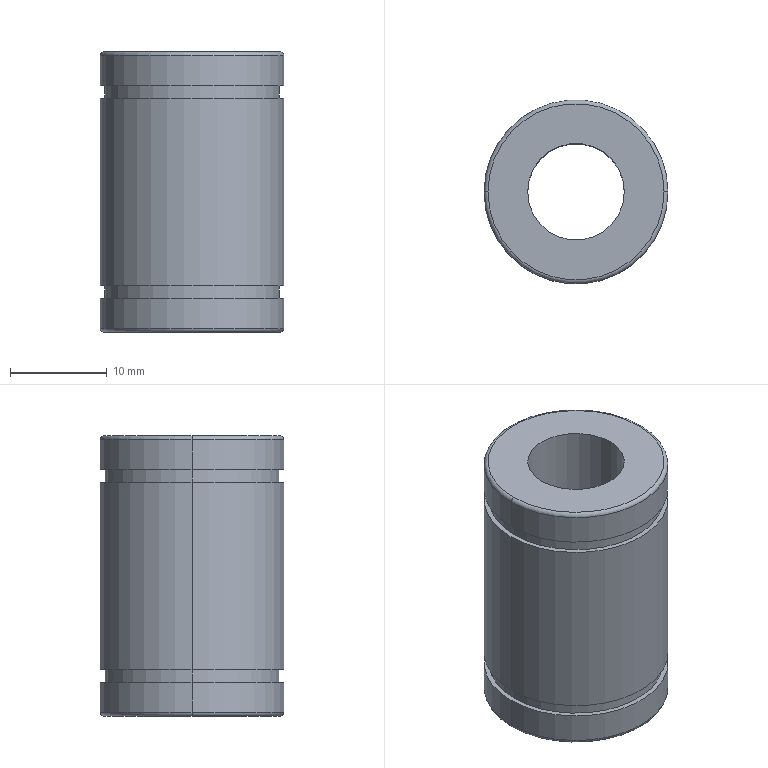Component | SolidWorks | LMU_N10-10 | 1 solid | 22 faces | box 19 x 19 x 29 mm | volume 5865 mm3 | cylinder 12 | plane 6 | torus 4 | commonest cylinder face diameters 19 x6 18 x4 10 x2
build123d program:
from build123d import *


with BuildPart() as part:
    # Sketch1 → Revolve1 (revolve)
    with BuildSketch(Plane.XY, mode=Mode.PRIVATE) as revolve1_sk:
        with BuildLine():
            Line((0, 9.1), (0, 5))
            Line((0, 5), (29, 5))
            Line((29, 5), (29, 9.1))
            ThreePointArc((29, 9.1), (28.883, 9.383), (28.6, 9.5))
            Line((28.6, 9.5), (25.5, 9.5))
            Line((25.5, 9.5), (25.5, 9))
            Line((25.5, 9), (24.2, 9))
            Line((24.2, 9), (24.2, 9.5))
            Line((24.2, 9.5), (4.8, 9.5))
            Line((4.8, 9.5), (4.8, 9))
            Line((4.8, 9), (3.5, 9))
            Line((3.5, 9), (3.5, 9.5))
            Line((3.5, 9.5), (0.4, 9.5))
            ThreePointArc((0.4, 9.5), (0.1172, 9.383), (0, 9.1))
        make_face()
    revolve(revolve1_sk.sketch.rotate(Axis((29, 0, 0), (-1, 0, 0)), 270), axis=Axis((29, 0, 0), (-1, 0, 0)))


solid = part.part

# Placed as in the assembly
solid = solid.moved(Location((860.265, 384.385, -295.193), (0, 90, 0)))
STEP:
#1=COLOUR_RGB('',0.7922,0.8196,0.9333);
#2=FILL_AREA_STYLE_COLOUR('',#1);
#3=FILL_AREA_STYLE('',(#2));
#4=SURFACE_STYLE_FILL_AREA(#3);
#5=SURFACE_SIDE_STYLE('',(#4));
#6=SURFACE_STYLE_USAGE(.BOTH.,#5);
#7=PRESENTATION_STYLE_ASSIGNMENT((#6));
#8=CARTESIAN_POINT('',(33.495,15.133,-12.626));
#9=VERTEX_POINT('',#8);
#10=CARTESIAN_POINT('',(34.243,15.133,-12.626));
#11=VERTEX_POINT('',#10);
#12=CARTESIAN_POINT('',(33.869,15.133,-12.626));
#13=DIRECTION('',(-0.00002551,-0.,-1.));
#14=DIRECTION('',(-1.,0.,0.00002551));
#15=AXIS2_PLACEMENT_3D('',#12,#13,#14);
#16=CIRCLE('',#15,0.374);
#17=EDGE_CURVE('',#9,#11,#16,.T.);
#18=ORIENTED_EDGE('',*,*,#17,.T.);
#19=CARTESIAN_POINT('',(34.243,15.133,-12.748));
#20=VERTEX_POINT('',#19);
#21=CARTESIAN_POINT('',(34.243,15.133,-11.622));
#22=DIRECTION('',(-0.00002551,-0.,-1.));
#23=VECTOR('',#22,39.37);
#24=LINE('',#21,#23);
#25=EDGE_CURVE('',#11,#20,#24,.T.);
#26=ORIENTED_EDGE('',*,*,#25,.T.);
#27=CARTESIAN_POINT('',(33.495,15.133,-12.748));
#28=VERTEX_POINT('',#27);
#29=CARTESIAN_POINT('',(33.869,15.133,-12.748));
#30=DIRECTION('',(-0.00002551,-0.,-1.));
#31=DIRECTION('',(-1.,0.,0.00002551));
#32=AXIS2_PLACEMENT_3D('',#29,#30,#31);
#33=CIRCLE('',#32,0.374);
#34=EDGE_CURVE('',#28,#20,#33,.T.);
#35=ORIENTED_EDGE('',*,*,#34,.F.);
#36=CARTESIAN_POINT('',(33.495,15.133,-11.622));
#37=DIRECTION('',(-0.00002551,-0.,-1.));
#38=VECTOR('',#37,39.37);
#39=LINE('',#36,#38);
#40=EDGE_CURVE('',#9,#28,#39,.T.);
#41=ORIENTED_EDGE('',*,*,#40,.F.);
#42=EDGE_LOOP('',(#18,#26,#35,#41));
#43=FACE_OUTER_BOUND('',#42,.T.);
#44=CARTESIAN_POINT('',(33.869,15.133,-11.622));
#45=DIRECTION('',(-0.00002551,-0.,-1.));
#46=DIRECTION('',(-1.,0.,0.00002551));
#47=AXIS2_PLACEMENT_3D('',#44,#45,#46);
#48=CYLINDRICAL_SURFACE('',#47,0.374);
#49=ADVANCED_FACE('',(#43),#48,.T.);
#50=CARTESIAN_POINT('',(33.514,15.133,-12.575));
#51=VERTEX_POINT('',#50);
#52=CARTESIAN_POINT('',(34.223,15.133,-12.575));
#53=VERTEX_POINT('',#52);
#54=CARTESIAN_POINT('',(33.869,15.133,-12.575));
#55=DIRECTION('',(-0.00002551,-0.,-1.));
#56=DIRECTION('',(-1.,0.,0.00002551));
#57=AXIS2_PLACEMENT_3D('',#54,#55,#56);
#58=CIRCLE('',#57,0.3543);
#59=EDGE_CURVE('',#51,#53,#58,.T.);
#60=ORIENTED_EDGE('',*,*,#59,.T.);
#61=CARTESIAN_POINT('',(34.223,15.133,-12.626));
#62=VERTEX_POINT('',#61);
#63=CARTESIAN_POINT('',(34.223,15.133,-11.622));
#64=DIRECTION('',(-0.00002551,-0.,-1.));
#65=VECTOR('',#64,39.37);
#66=LINE('',#63,#65);
#67=EDGE_CURVE('',#53,#62,#66,.T.);
#68=ORIENTED_EDGE('',*,*,#67,.T.);
#69=CARTESIAN_POINT('',(33.514,15.133,-12.626));
#70=VERTEX_POINT('',#69);
#71=CARTESIAN_POINT('',(33.869,15.133,-12.626));
#72=DIRECTION('',(-0.00002551,-0.,-1.));
#73=DIRECTION('',(-1.,0.,0.00002551));
#74=AXIS2_PLACEMENT_3D('',#71,#72,#73);
#75=CIRCLE('',#74,0.3543);
#76=EDGE_CURVE('',#70,#62,#75,.T.);
#77=ORIENTED_EDGE('',*,*,#76,.F.);
#78=CARTESIAN_POINT('',(33.514,15.133,-11.622));
#79=DIRECTION('',(-0.00002551,-0.,-1.));
#80=VECTOR('',#79,39.37);
#81=LINE('',#78,#80);
#82=EDGE_CURVE('',#51,#70,#81,.T.);
#83=ORIENTED_EDGE('',*,*,#82,.F.);
#84=EDGE_LOOP('',(#60,#68,#77,#83));
#85=FACE_OUTER_BOUND('',#84,.T.);
#86=CARTESIAN_POINT('',(33.869,15.133,-11.622));
#87=DIRECTION('',(-0.00002551,-0.,-1.));
#88=DIRECTION('',(-1.,0.,0.00002551));
#89=AXIS2_PLACEMENT_3D('',#86,#87,#88);
#90=CYLINDRICAL_SURFACE('',#89,0.3543);
#91=ADVANCED_FACE('',(#85),#90,.T.);
#92=CARTESIAN_POINT('',(33.495,15.133,-11.811));
#93=VERTEX_POINT('',#92);
#94=CARTESIAN_POINT('',(34.243,15.133,-11.811));
#95=VERTEX_POINT('',#94);
#96=CARTESIAN_POINT('',(33.869,15.133,-11.811));
#97=DIRECTION('',(-0.00002551,-0.,-1.));
#98=DIRECTION('',(-1.,0.,0.00002551));
#99=AXIS2_PLACEMENT_3D('',#96,#97,#98);
#100=CIRCLE('',#99,0.374);
#101=EDGE_CURVE('',#93,#95,#100,.T.);
#102=ORIENTED_EDGE('',*,*,#101,.T.);
#103=CARTESIAN_POINT('',(34.243,15.133,-12.575));
#104=VERTEX_POINT('',#103);
#105=CARTESIAN_POINT('',(34.243,15.133,-11.622));
#106=DIRECTION('',(-0.00002551,-0.,-1.));
#107=VECTOR('',#106,39.37);
#108=LINE('',#105,#107);
#109=EDGE_CURVE('',#95,#104,#108,.T.);
#110=ORIENTED_EDGE('',*,*,#109,.T.);
#111=CARTESIAN_POINT('',(33.495,15.133,-12.575));
#112=VERTEX_POINT('',#111);
#113=CARTESIAN_POINT('',(33.869,15.133,-12.575));
#114=DIRECTION('',(-0.00002551,-0.,-1.));
#115=DIRECTION('',(-1.,0.,0.00002551));
#116=AXIS2_PLACEMENT_3D('',#113,#114,#115);
#117=CIRCLE('',#116,0.374);
#118=EDGE_CURVE('',#112,#104,#117,.T.);
#119=ORIENTED_EDGE('',*,*,#118,.F.);
#120=CARTESIAN_POINT('',(33.495,15.133,-11.622));
#121=DIRECTION('',(-0.00002551,-0.,-1.));
#122=VECTOR('',#121,39.37);
#123=LINE('',#120,#122);
#124=EDGE_CURVE('',#93,#112,#123,.T.);
#125=ORIENTED_EDGE('',*,*,#124,.F.);
#126=EDGE_LOOP('',(#102,#110,#119,#125));
#127=FACE_OUTER_BOUND('',#126,.T.);
#128=CARTESIAN_POINT('',(33.869,15.133,-11.622));
#129=DIRECTION('',(-0.00002551,-0.,-1.));
#130=DIRECTION('',(-1.,0.,0.00002551));
#131=AXIS2_PLACEMENT_3D('',#128,#129,#130);
#132=CYLINDRICAL_SURFACE('',#131,0.374);
#133=ADVANCED_FACE('',(#127),#132,.T.);
#134=CARTESIAN_POINT('',(33.514,15.133,-11.76));
#135=VERTEX_POINT('',#134);
#136=CARTESIAN_POINT('',(34.223,15.133,-11.76));
#137=VERTEX_POINT('',#136);
#138=CARTESIAN_POINT('',(33.869,15.133,-11.76));
#139=DIRECTION('',(-0.00002551,-0.,-1.));
#140=DIRECTION('',(-1.,0.,0.00002551));
#141=AXIS2_PLACEMENT_3D('',#138,#139,#140);
#142=CIRCLE('',#141,0.3543);
#143=EDGE_CURVE('',#135,#137,#142,.T.);
#144=ORIENTED_EDGE('',*,*,#143,.T.);
#145=CARTESIAN_POINT('',(34.223,15.133,-11.811));
#146=VERTEX_POINT('',#145);
#147=CARTESIAN_POINT('',(34.223,15.133,-11.622));
#148=DIRECTION('',(-0.00002551,-0.,-1.));
#149=VECTOR('',#148,39.37);
#150=LINE('',#147,#149);
#151=EDGE_CURVE('',#137,#146,#150,.T.);
#152=ORIENTED_EDGE('',*,*,#151,.T.);
#153=CARTESIAN_POINT('',(33.514,15.133,-11.811));
#154=VERTEX_POINT('',#153);
#155=CARTESIAN_POINT('',(33.869,15.133,-11.811));
#156=DIRECTION('',(-0.00002551,-0.,-1.));
#157=DIRECTION('',(-1.,0.,0.00002551));
#158=AXIS2_PLACEMENT_3D('',#155,#156,#157);
#159=CIRCLE('',#158,0.3543);
#160=EDGE_CURVE('',#154,#146,#159,.T.);
#161=ORIENTED_EDGE('',*,*,#160,.F.);
#162=CARTESIAN_POINT('',(33.514,15.133,-11.622));
#163=DIRECTION('',(-0.00002551,-0.,-1.));
#164=VECTOR('',#163,39.37);
#165=LINE('',#162,#164);
#166=EDGE_CURVE('',#135,#154,#165,.T.);
#167=ORIENTED_EDGE('',*,*,#166,.F.);
#168=EDGE_LOOP('',(#144,#152,#161,#167));
#169=FACE_OUTER_BOUND('',#168,.T.);
#170=CARTESIAN_POINT('',(33.869,15.133,-11.622));
#171=DIRECTION('',(-0.00002551,-0.,-1.));
#172=DIRECTION('',(-1.,0.,0.00002551));
#173=AXIS2_PLACEMENT_3D('',#170,#171,#172);
#174=CYLINDRICAL_SURFACE('',#173,0.3543);
#175=ADVANCED_FACE('',(#169),#174,.T.);
#176=CARTESIAN_POINT('',(33.495,15.133,-11.638));
#177=VERTEX_POINT('',#176);
#178=CARTESIAN_POINT('',(34.243,15.133,-11.638));
#179=VERTEX_POINT('',#178);
#180=CARTESIAN_POINT('',(33.869,15.133,-11.638));
#181=DIRECTION('',(-0.00002551,-0.,-1.));
#182=DIRECTION('',(-1.,0.,0.00002551));
#183=AXIS2_PLACEMENT_3D('',#180,#181,#182);
#184=CIRCLE('',#183,0.374);
#185=EDGE_CURVE('',#177,#179,#184,.T.);
#186=ORIENTED_EDGE('',*,*,#185,.T.);
#187=CARTESIAN_POINT('',(34.243,15.133,-11.76));
#188=VERTEX_POINT('',#187);
#189=CARTESIAN_POINT('',(34.243,15.133,-11.622));
#190=DIRECTION('',(-0.00002551,-0.,-1.));
#191=VECTOR('',#190,39.37);
#192=LINE('',#189,#191);
#193=EDGE_CURVE('',#179,#188,#192,.T.);
#194=ORIENTED_EDGE('',*,*,#193,.T.);
#195=CARTESIAN_POINT('',(33.495,15.133,-11.76));
#196=VERTEX_POINT('',#195);
#197=CARTESIAN_POINT('',(33.869,15.133,-11.76));
#198=DIRECTION('',(-0.00002551,-0.,-1.));
#199=DIRECTION('',(-1.,0.,0.00002551));
#200=AXIS2_PLACEMENT_3D('',#197,#198,#199);
#201=CIRCLE('',#200,0.374);
#202=EDGE_CURVE('',#196,#188,#201,.T.);
#203=ORIENTED_EDGE('',*,*,#202,.F.);
#204=CARTESIAN_POINT('',(33.495,15.133,-11.622));
#205=DIRECTION('',(-0.00002551,-0.,-1.));
#206=VECTOR('',#205,39.37);
#207=LINE('',#204,#206);
#208=EDGE_CURVE('',#177,#196,#207,.T.);
#209=ORIENTED_EDGE('',*,*,#208,.F.);
#210=EDGE_LOOP('',(#186,#194,#203,#209));
#211=FACE_OUTER_BOUND('',#210,.T.);
#212=CARTESIAN_POINT('',(33.869,15.133,-11.622));
#213=DIRECTION('',(-0.00002551,-0.,-1.));
#214=DIRECTION('',(-1.,0.,0.00002551));
#215=AXIS2_PLACEMENT_3D('',#212,#213,#214);
#216=CYLINDRICAL_SURFACE('',#215,0.374);
#217=ADVANCED_FACE('',(#211),#216,.T.);
#218=CARTESIAN_POINT('',(33.51,15.133,-11.622));
#219=VERTEX_POINT('',#218);
#220=CARTESIAN_POINT('',(34.227,15.133,-11.622));
#221=VERTEX_POINT('',#220);
#222=CARTESIAN_POINT('',(33.869,15.133,-11.622));
#223=DIRECTION('',(-0.00002551,-0.,-1.));
#224=DIRECTION('',(-1.,0.,0.00002551));
#225=AXIS2_PLACEMENT_3D('',#222,#223,#224);
#226=CIRCLE('',#225,0.3583);
#227=EDGE_CURVE('',#219,#221,#226,.T.);
#228=ORIENTED_EDGE('',*,*,#227,.T.);
#229=CARTESIAN_POINT('',(34.227,15.133,-11.638));
#230=DIRECTION('',(-0.,1.,-0.));
#231=DIRECTION('',(-1.,0.,0.));
#232=AXIS2_PLACEMENT_3D('',#229,#230,#231);
#233=CIRCLE('',#232,0.01575);
#234=EDGE_CURVE('',#221,#179,#233,.T.);
#235=ORIENTED_EDGE('',*,*,#234,.T.);
#236=ORIENTED_EDGE('',*,*,#185,.F.);
#237=CARTESIAN_POINT('',(33.51,15.133,-11.638));
#238=DIRECTION('',(0.,-1.,0.));
#239=DIRECTION('',(1.,0.,0.));
#240=AXIS2_PLACEMENT_3D('',#237,#238,#239);
#241=CIRCLE('',#240,0.01575);
#242=EDGE_CURVE('',#219,#177,#241,.T.);
#243=ORIENTED_EDGE('',*,*,#242,.F.);
#244=EDGE_LOOP('',(#228,#235,#236,#243));
#245=FACE_OUTER_BOUND('',#244,.T.);
#246=CARTESIAN_POINT('',(33.869,15.133,-11.638));
#247=DIRECTION('',(-0.00002551,-0.,-1.));
#248=DIRECTION('',(-1.,-0.,0.00002551));
#249=AXIS2_PLACEMENT_3D('',#246,#247,#248);
#250=TOROIDAL_SURFACE('',#249,0.3583,0.01575);
#251=ADVANCED_FACE('',(#245),#250,.T.);
#252=CARTESIAN_POINT('',(34.066,15.133,-11.622));
#253=VERTEX_POINT('',#252);
#254=CARTESIAN_POINT('',(33.672,15.133,-11.622));
#255=VERTEX_POINT('',#254);
#256=CARTESIAN_POINT('',(33.869,15.133,-11.622));
#257=DIRECTION('',(-0.00002551,-0.,-1.));
#258=DIRECTION('',(-1.,0.,0.00002551));
#259=AXIS2_PLACEMENT_3D('',#256,#257,#258);
#260=CIRCLE('',#259,0.1969);
#261=EDGE_CURVE('',#253,#255,#260,.T.);
#262=ORIENTED_EDGE('',*,*,#261,.F.);
#263=CARTESIAN_POINT('',(34.066,15.133,-12.764));
#264=VERTEX_POINT('',#263);
#265=CARTESIAN_POINT('',(34.066,15.133,-11.622));
#266=DIRECTION('',(-0.00002551,-0.,-1.));
#267=VECTOR('',#266,39.37);
#268=LINE('',#265,#267);
#269=EDGE_CURVE('',#253,#264,#268,.T.);
#270=ORIENTED_EDGE('',*,*,#269,.T.);
#271=CARTESIAN_POINT('',(33.672,15.133,-12.764));
#272=VERTEX_POINT('',#271);
#273=CARTESIAN_POINT('',(33.869,15.133,-12.764));
#274=DIRECTION('',(-0.00002551,-0.,-1.));
#275=DIRECTION('',(-1.,0.,0.00002551));
#276=AXIS2_PLACEMENT_3D('',#273,#274,#275);
#277=CIRCLE('',#276,0.1969);
#278=EDGE_CURVE('',#264,#272,#277,.T.);
#279=ORIENTED_EDGE('',*,*,#278,.T.);
#280=CARTESIAN_POINT('',(33.672,15.133,-11.622));
#281=DIRECTION('',(-0.00002551,-0.,-1.));
#282=VECTOR('',#281,39.37);
#283=LINE('',#280,#282);
#284=EDGE_CURVE('',#255,#272,#283,.T.);
#285=ORIENTED_EDGE('',*,*,#284,.F.);
#286=EDGE_LOOP('',(#262,#270,#279,#285));
#287=FACE_OUTER_BOUND('',#286,.T.);
#288=CARTESIAN_POINT('',(33.869,15.133,-11.622));
#289=DIRECTION('',(-0.00002551,-0.,-1.));
#290=DIRECTION('',(-1.,0.,0.00002551));
#291=AXIS2_PLACEMENT_3D('',#288,#289,#290);
#292=CYLINDRICAL_SURFACE('',#291,0.1969);
#293=ADVANCED_FACE('',(#287),#292,.F.);
#294=ORIENTED_EDGE('',*,*,#34,.T.);
#295=CARTESIAN_POINT('',(34.227,15.133,-12.764));
#296=VERTEX_POINT('',#295);
#297=CARTESIAN_POINT('',(34.227,15.133,-12.748));
#298=DIRECTION('',(-0.,1.,-0.));
#299=DIRECTION('',(-1.,0.,0.));
#300=AXIS2_PLACEMENT_3D('',#297,#298,#299);
#301=CIRCLE('',#300,0.01575);
#302=EDGE_CURVE('',#20,#296,#301,.T.);
#303=ORIENTED_EDGE('',*,*,#302,.T.);
#304=CARTESIAN_POINT('',(33.51,15.133,-12.764));
#305=VERTEX_POINT('',#304);
#306=CARTESIAN_POINT('',(33.869,15.133,-12.764));
#307=DIRECTION('',(-0.00002551,-0.,-1.));
#308=DIRECTION('',(-1.,0.,0.00002551));
#309=AXIS2_PLACEMENT_3D('',#306,#307,#308);
#310=CIRCLE('',#309,0.3583);
#311=EDGE_CURVE('',#305,#296,#310,.T.);
#312=ORIENTED_EDGE('',*,*,#311,.F.);
#313=CARTESIAN_POINT('',(33.51,15.133,-12.748));
#314=DIRECTION('',(0.,-1.,0.));
#315=DIRECTION('',(1.,0.,0.));
#316=AXIS2_PLACEMENT_3D('',#313,#314,#315);
#317=CIRCLE('',#316,0.01575);
#318=EDGE_CURVE('',#28,#305,#317,.T.);
#319=ORIENTED_EDGE('',*,*,#318,.F.);
#320=EDGE_LOOP('',(#294,#303,#312,#319));
#321=FACE_OUTER_BOUND('',#320,.T.);
#322=CARTESIAN_POINT('',(33.869,15.133,-12.748));
#323=DIRECTION('',(-0.00002551,-0.,-1.));
#324=DIRECTION('',(-1.,-0.,0.00002551));
#325=AXIS2_PLACEMENT_3D('',#322,#323,#324);
#326=TOROIDAL_SURFACE('',#325,0.3583,0.01575);
#327=ADVANCED_FACE('',(#321),#326,.T.);
#328=ORIENTED_EDGE('',*,*,#302,.F.);
#329=CARTESIAN_POINT('',(33.869,15.133,-12.748));
#330=DIRECTION('',(-0.00002551,-0.,-1.));
#331=DIRECTION('',(-1.,0.,0.00002551));
#332=AXIS2_PLACEMENT_3D('',#329,#330,#331);
#333=CIRCLE('',#332,0.374);
#334=EDGE_CURVE('',#20,#28,#333,.T.);
#335=ORIENTED_EDGE('',*,*,#334,.T.);
#336=ORIENTED_EDGE('',*,*,#318,.T.);
#337=CARTESIAN_POINT('',(33.869,15.133,-12.764));
#338=DIRECTION('',(-0.00002551,-0.,-1.));
#339=DIRECTION('',(-1.,0.,0.00002551));
#340=AXIS2_PLACEMENT_3D('',#337,#338,#339);
#341=CIRCLE('',#340,0.3583);
#342=EDGE_CURVE('',#296,#305,#341,.T.);
#343=ORIENTED_EDGE('',*,*,#342,.F.);
#344=EDGE_LOOP('',(#328,#335,#336,#343));
#345=FACE_OUTER_BOUND('',#344,.T.);
#346=CARTESIAN_POINT('',(33.869,15.133,-12.748));
#347=DIRECTION('',(-0.00002551,-0.,-1.));
#348=DIRECTION('',(-1.,-0.,0.00002551));
#349=AXIS2_PLACEMENT_3D('',#346,#347,#348);
#350=TOROIDAL_SURFACE('',#349,0.3583,0.01575);
#351=ADVANCED_FACE('',(#345),#350,.T.);
#352=CARTESIAN_POINT('',(33.869,15.133,-12.764));
#353=DIRECTION('',(-0.00002551,-0.,-1.));
#354=DIRECTION('',(-1.,0.,0.00002551));
#355=AXIS2_PLACEMENT_3D('',#352,#353,#354);
#356=CIRCLE('',#355,0.1969);
#357=EDGE_CURVE('',#272,#264,#356,.T.);
#358=ORIENTED_EDGE('',*,*,#357,.F.);
#359=ORIENTED_EDGE('',*,*,#278,.F.);
#360=EDGE_LOOP('',(#358,#359));
#361=FACE_BOUND('',#360,.T.);
#362=ORIENTED_EDGE('',*,*,#311,.T.);
#363=ORIENTED_EDGE('',*,*,#342,.T.);
#364=EDGE_LOOP('',(#362,#363));
#365=FACE_OUTER_BOUND('',#364,.T.);
#366=CARTESIAN_POINT('',(33.869,15.492,-12.764));
#367=DIRECTION('',(0.00002551,0.,1.));
#368=DIRECTION('',(1.,0.,-0.00002551));
#369=AXIS2_PLACEMENT_3D('',#366,#367,#368);
#370=PLANE('',#369);
#371=ADVANCED_FACE('',(#361,#365),#370,.F.);
#372=ORIENTED_EDGE('',*,*,#269,.F.);
#373=CARTESIAN_POINT('',(33.869,15.133,-11.622));
#374=DIRECTION('',(-0.00002551,-0.,-1.));
#375=DIRECTION('',(-1.,0.,0.00002551));
#376=AXIS2_PLACEMENT_3D('',#373,#374,#375);
#377=CIRCLE('',#376,0.1969);
#378=EDGE_CURVE('',#255,#253,#377,.T.);
#379=ORIENTED_EDGE('',*,*,#378,.F.);
#380=ORIENTED_EDGE('',*,*,#284,.T.);
#381=ORIENTED_EDGE('',*,*,#357,.T.);
#382=EDGE_LOOP('',(#372,#379,#380,#381));
#383=FACE_OUTER_BOUND('',#382,.T.);
#384=CARTESIAN_POINT('',(33.869,15.133,-11.622));
#385=DIRECTION('',(-0.00002551,-0.,-1.));
#386=DIRECTION('',(-1.,0.,0.00002551));
#387=AXIS2_PLACEMENT_3D('',#384,#385,#386);
#388=CYLINDRICAL_SURFACE('',#387,0.1969);
#389=ADVANCED_FACE('',(#383),#388,.F.);
#390=ORIENTED_EDGE('',*,*,#227,.F.);
#391=CARTESIAN_POINT('',(33.869,15.133,-11.622));
#392=DIRECTION('',(-0.00002551,-0.,-1.));
#393=DIRECTION('',(-1.,0.,0.00002551));
#394=AXIS2_PLACEMENT_3D('',#391,#392,#393);
#395=CIRCLE('',#394,0.3583);
#396=EDGE_CURVE('',#221,#219,#395,.T.);
#397=ORIENTED_EDGE('',*,*,#396,.F.);
#398=EDGE_LOOP('',(#390,#397));
#399=FACE_OUTER_BOUND('',#398,.T.);
#400=ORIENTED_EDGE('',*,*,#378,.T.);
#401=ORIENTED_EDGE('',*,*,#261,.T.);
#402=EDGE_LOOP('',(#400,#401));
#403=FACE_BOUND('',#402,.T.);
#404=CARTESIAN_POINT('',(33.869,15.33,-11.622));
#405=DIRECTION('',(-0.00002551,-0.,-1.));
#406=DIRECTION('',(-1.,-0.,0.00002551));
#407=AXIS2_PLACEMENT_3D('',#404,#405,#406);
#408=PLANE('',#407);
#409=ADVANCED_FACE('',(#399,#403),#408,.F.);
#410=ORIENTED_EDGE('',*,*,#234,.F.);
#411=ORIENTED_EDGE('',*,*,#396,.T.);
#412=ORIENTED_EDGE('',*,*,#242,.T.);
#413=CARTESIAN_POINT('',(33.869,15.133,-11.638));
#414=DIRECTION('',(-0.00002551,-0.,-1.));
#415=DIRECTION('',(-1.,0.,0.00002551));
#416=AXIS2_PLACEMENT_3D('',#413,#414,#415);
#417=CIRCLE('',#416,0.374);
#418=EDGE_CURVE('',#179,#177,#417,.T.);
#419=ORIENTED_EDGE('',*,*,#418,.F.);
#420=EDGE_LOOP('',(#410,#411,#412,#419));
#421=FACE_OUTER_BOUND('',#420,.T.);
#422=CARTESIAN_POINT('',(33.869,15.133,-11.638));
#423=DIRECTION('',(-0.00002551,-0.,-1.));
#424=DIRECTION('',(-1.,-0.,0.00002551));
#425=AXIS2_PLACEMENT_3D('',#422,#423,#424);
#426=TOROIDAL_SURFACE('',#425,0.3583,0.01575);
#427=ADVANCED_FACE('',(#421),#426,.T.);
#428=ORIENTED_EDGE('',*,*,#193,.F.);
#429=ORIENTED_EDGE('',*,*,#418,.T.);
#430=ORIENTED_EDGE('',*,*,#208,.T.);
#431=CARTESIAN_POINT('',(33.869,15.133,-11.76));
#432=DIRECTION('',(-0.00002551,-0.,-1.));
#433=DIRECTION('',(-1.,0.,0.00002551));
#434=AXIS2_PLACEMENT_3D('',#431,#432,#433);
#435=CIRCLE('',#434,0.374);
#436=EDGE_CURVE('',#188,#196,#435,.T.);
#437=ORIENTED_EDGE('',*,*,#436,.F.);
#438=EDGE_LOOP('',(#428,#429,#430,#437));
#439=FACE_OUTER_BOUND('',#438,.T.);
#440=CARTESIAN_POINT('',(33.869,15.133,-11.622));
#441=DIRECTION('',(-0.00002551,-0.,-1.));
#442=DIRECTION('',(-1.,0.,0.00002551));
#443=AXIS2_PLACEMENT_3D('',#440,#441,#442);
#444=CYLINDRICAL_SURFACE('',#443,0.374);
#445=ADVANCED_FACE('',(#439),#444,.T.);
#446=ORIENTED_EDGE('',*,*,#143,.F.);
#447=CARTESIAN_POINT('',(33.869,15.133,-11.76));
#448=DIRECTION('',(-0.00002551,-0.,-1.));
#449=DIRECTION('',(-1.,0.,0.00002551));
#450=AXIS2_PLACEMENT_3D('',#447,#448,#449);
#451=CIRCLE('',#450,0.3543);
#452=EDGE_CURVE('',#137,#135,#451,.T.);
#453=ORIENTED_EDGE('',*,*,#452,.F.);
#454=EDGE_LOOP('',(#446,#453));
#455=FACE_BOUND('',#454,.T.);
#456=ORIENTED_EDGE('',*,*,#202,.T.);
#457=ORIENTED_EDGE('',*,*,#436,.T.);
#458=EDGE_LOOP('',(#456,#457));
#459=FACE_OUTER_BOUND('',#458,.T.);
#460=CARTESIAN_POINT('',(33.869,15.507,-11.76));
#461=DIRECTION('',(0.00002551,0.,1.));
#462=DIRECTION('',(1.,0.,-0.00002551));
#463=AXIS2_PLACEMENT_3D('',#460,#461,#462);
#464=PLANE('',#463);
#465=ADVANCED_FACE('',(#455,#459),#464,.F.);
#466=ORIENTED_EDGE('',*,*,#151,.F.);
#467=ORIENTED_EDGE('',*,*,#452,.T.);
#468=ORIENTED_EDGE('',*,*,#166,.T.);
#469=CARTESIAN_POINT('',(33.869,15.133,-11.811));
#470=DIRECTION('',(-0.00002551,-0.,-1.));
#471=DIRECTION('',(-1.,0.,0.00002551));
#472=AXIS2_PLACEMENT_3D('',#469,#470,#471);
#473=CIRCLE('',#472,0.3543);
#474=EDGE_CURVE('',#146,#154,#473,.T.);
#475=ORIENTED_EDGE('',*,*,#474,.F.);
#476=EDGE_LOOP('',(#466,#467,#468,#475));
#477=FACE_OUTER_BOUND('',#476,.T.);
#478=CARTESIAN_POINT('',(33.869,15.133,-11.622));
#479=DIRECTION('',(-0.00002551,-0.,-1.));
#480=DIRECTION('',(-1.,0.,0.00002551));
#481=AXIS2_PLACEMENT_3D('',#478,#479,#480);
#482=CYLINDRICAL_SURFACE('',#481,0.3543);
#483=ADVANCED_FACE('',(#477),#482,.T.);
#484=ORIENTED_EDGE('',*,*,#101,.F.);
#485=CARTESIAN_POINT('',(33.869,15.133,-11.811));
#486=DIRECTION('',(-0.00002551,-0.,-1.));
#487=DIRECTION('',(-1.,0.,0.00002551));
#488=AXIS2_PLACEMENT_3D('',#485,#486,#487);
#489=CIRCLE('',#488,0.374);
#490=EDGE_CURVE('',#95,#93,#489,.T.);
#491=ORIENTED_EDGE('',*,*,#490,.F.);
#492=EDGE_LOOP('',(#484,#491));
#493=FACE_OUTER_BOUND('',#492,.T.);
#494=ORIENTED_EDGE('',*,*,#160,.T.);
#495=ORIENTED_EDGE('',*,*,#474,.T.);
#496=EDGE_LOOP('',(#494,#495));
#497=FACE_BOUND('',#496,.T.);
#498=CARTESIAN_POINT('',(33.869,15.488,-11.811));
#499=DIRECTION('',(-0.00002551,-0.,-1.));
#500=DIRECTION('',(-1.,-0.,0.00002551));
#501=AXIS2_PLACEMENT_3D('',#498,#499,#500);
#502=PLANE('',#501);
#503=ADVANCED_FACE('',(#493,#497),#502,.F.);
#504=ORIENTED_EDGE('',*,*,#109,.F.);
#505=ORIENTED_EDGE('',*,*,#490,.T.);
#506=ORIENTED_EDGE('',*,*,#124,.T.);
#507=CARTESIAN_POINT('',(33.869,15.133,-12.575));
#508=DIRECTION('',(-0.00002551,-0.,-1.));
#509=DIRECTION('',(-1.,0.,0.00002551));
#510=AXIS2_PLACEMENT_3D('',#507,#508,#509);
#511=CIRCLE('',#510,0.374);
#512=EDGE_CURVE('',#104,#112,#511,.T.);
#513=ORIENTED_EDGE('',*,*,#512,.F.);
#514=EDGE_LOOP('',(#504,#505,#506,#513));
#515=FACE_OUTER_BOUND('',#514,.T.);
#516=CARTESIAN_POINT('',(33.869,15.133,-11.622));
#517=DIRECTION('',(-0.00002551,-0.,-1.));
#518=DIRECTION('',(-1.,0.,0.00002551));
#519=AXIS2_PLACEMENT_3D('',#516,#517,#518);
#520=CYLINDRICAL_SURFACE('',#519,0.374);
#521=ADVANCED_FACE('',(#515),#520,.T.);
#522=ORIENTED_EDGE('',*,*,#59,.F.);
#523=CARTESIAN_POINT('',(33.869,15.133,-12.575));
#524=DIRECTION('',(-0.00002551,-0.,-1.));
#525=DIRECTION('',(-1.,0.,0.00002551));
#526=AXIS2_PLACEMENT_3D('',#523,#524,#525);
#527=CIRCLE('',#526,0.3543);
#528=EDGE_CURVE('',#53,#51,#527,.T.);
#529=ORIENTED_EDGE('',*,*,#528,.F.);
#530=EDGE_LOOP('',(#522,#529));
#531=FACE_BOUND('',#530,.T.);
#532=ORIENTED_EDGE('',*,*,#118,.T.);
#533=ORIENTED_EDGE('',*,*,#512,.T.);
#534=EDGE_LOOP('',(#532,#533));
#535=FACE_OUTER_BOUND('',#534,.T.);
#536=CARTESIAN_POINT('',(33.869,15.507,-12.575));
#537=DIRECTION('',(0.00002551,0.,1.));
#538=DIRECTION('',(1.,0.,-0.00002551));
#539=AXIS2_PLACEMENT_3D('',#536,#537,#538);
#540=PLANE('',#539);
#541=ADVANCED_FACE('',(#531,#535),#540,.F.);
#542=ORIENTED_EDGE('',*,*,#67,.F.);
#543=ORIENTED_EDGE('',*,*,#528,.T.);
#544=ORIENTED_EDGE('',*,*,#82,.T.);
#545=CARTESIAN_POINT('',(33.869,15.133,-12.626));
#546=DIRECTION('',(-0.00002551,-0.,-1.));
#547=DIRECTION('',(-1.,0.,0.00002551));
#548=AXIS2_PLACEMENT_3D('',#545,#546,#547);
#549=CIRCLE('',#548,0.3543);
#550=EDGE_CURVE('',#62,#70,#549,.T.);
#551=ORIENTED_EDGE('',*,*,#550,.F.);
#552=EDGE_LOOP('',(#542,#543,#544,#551));
#553=FACE_OUTER_BOUND('',#552,.T.);
#554=CARTESIAN_POINT('',(33.869,15.133,-11.622));
#555=DIRECTION('',(-0.00002551,-0.,-1.));
#556=DIRECTION('',(-1.,0.,0.00002551));
#557=AXIS2_PLACEMENT_3D('',#554,#555,#556);
#558=CYLINDRICAL_SURFACE('',#557,0.3543);
#559=ADVANCED_FACE('',(#553),#558,.T.);
#560=ORIENTED_EDGE('',*,*,#17,.F.);
#561=CARTESIAN_POINT('',(33.869,15.133,-12.626));
#562=DIRECTION('',(-0.00002551,-0.,-1.));
#563=DIRECTION('',(-1.,0.,0.00002551));
#564=AXIS2_PLACEMENT_3D('',#561,#562,#563);
#565=CIRCLE('',#564,0.374);
#566=EDGE_CURVE('',#11,#9,#565,.T.);
#567=ORIENTED_EDGE('',*,*,#566,.F.);
#568=EDGE_LOOP('',(#560,#567));
#569=FACE_OUTER_BOUND('',#568,.T.);
#570=ORIENTED_EDGE('',*,*,#76,.T.);
#571=ORIENTED_EDGE('',*,*,#550,.T.);
#572=EDGE_LOOP('',(#570,#571));
#573=FACE_BOUND('',#572,.T.);
#574=CARTESIAN_POINT('',(33.869,15.488,-12.626));
#575=DIRECTION('',(-0.00002551,-0.,-1.));
#576=DIRECTION('',(-1.,-0.,0.00002551));
#577=AXIS2_PLACEMENT_3D('',#574,#575,#576);
#578=PLANE('',#577);
#579=ADVANCED_FACE('',(#569,#573),#578,.F.);
#580=ORIENTED_EDGE('',*,*,#25,.F.);
#581=ORIENTED_EDGE('',*,*,#566,.T.);
#582=ORIENTED_EDGE('',*,*,#40,.T.);
#583=ORIENTED_EDGE('',*,*,#334,.F.);
#584=EDGE_LOOP('',(#580,#581,#582,#583));
#585=FACE_OUTER_BOUND('',#584,.T.);
#586=CARTESIAN_POINT('',(33.869,15.133,-11.622));
#587=DIRECTION('',(-0.00002551,-0.,-1.));
#588=DIRECTION('',(-1.,0.,0.00002551));
#589=AXIS2_PLACEMENT_3D('',#586,#587,#588);
#590=CYLINDRICAL_SURFACE('',#589,0.374);
#591=ADVANCED_FACE('',(#585),#590,.T.);
#592=CLOSED_SHELL('',(#49,#91,#133,#175,#217,#251,#293,#327,#351,#371,#389,#409,#427,#445,#465,#483,#503,#521,#541,#559,#579,#591));
#593=MANIFOLD_SOLID_BREP('',#592);
#594=STYLED_ITEM('',(#7),#593);
#595=(LENGTH_UNIT()NAMED_UNIT(*)SI_UNIT($,.METRE.));
#596=LENGTH_MEASURE_WITH_UNIT(LENGTH_MEASURE(0.0254),#595);
#597=DIMENSIONAL_EXPONENTS(1.,0.,0.,0.,0.,0.,0.);
#598=(CONVERSION_BASED_UNIT('',#596)LENGTH_UNIT()NAMED_UNIT(#597));
#599=UNCERTAINTY_MEASURE_WITH_UNIT(LENGTH_MEASURE(0.00001),#598,'','');
#600=(NAMED_UNIT(*)PLANE_ANGLE_UNIT()SI_UNIT($,.RADIAN.));
#601=(NAMED_UNIT(*)SI_UNIT($,.STERADIAN.)SOLID_ANGLE_UNIT());
#602=(GEOMETRIC_REPRESENTATION_CONTEXT(3)GLOBAL_UNCERTAINTY_ASSIGNED_CONTEXT((#599))GLOBAL_UNIT_ASSIGNED_CONTEXT((#598,#600,#601))REPRESENTATION_CONTEXT('',''));
#603=MECHANICAL_DESIGN_GEOMETRIC_PRESENTATION_REPRESENTATION('',(#594),#602);
#604=PRESENTATION_LAYER_ASSIGNMENT('','',(#594));
#605=CARTESIAN_POINT('',(0.,0.,0.));
#606=DIRECTION('',(0.,0.,1.));
#607=DIRECTION('',(1.,0.,0.));
#608=AXIS2_PLACEMENT_3D('',#605,#606,#607);
#609=(LENGTH_UNIT()NAMED_UNIT(*)SI_UNIT($,.METRE.));
#610=LENGTH_MEASURE_WITH_UNIT(LENGTH_MEASURE(0.0254),#609);
#611=DIMENSIONAL_EXPONENTS(1.,0.,0.,0.,0.,0.,0.);
#612=(CONVERSION_BASED_UNIT('',#610)LENGTH_UNIT()NAMED_UNIT(#611));
#613=UNCERTAINTY_MEASURE_WITH_UNIT(LENGTH_MEASURE(0.00001),#612,'','');
#614=(NAMED_UNIT(*)PLANE_ANGLE_UNIT()SI_UNIT($,.RADIAN.));
#615=(NAMED_UNIT(*)SI_UNIT($,.STERADIAN.)SOLID_ANGLE_UNIT());
#616=(GEOMETRIC_REPRESENTATION_CONTEXT(3)GLOBAL_UNCERTAINTY_ASSIGNED_CONTEXT((#613))GLOBAL_UNIT_ASSIGNED_CONTEXT((#612,#614,#615))REPRESENTATION_CONTEXT('',''));
#617=ADVANCED_BREP_SHAPE_REPRESENTATION('',(#593,#608),#616);